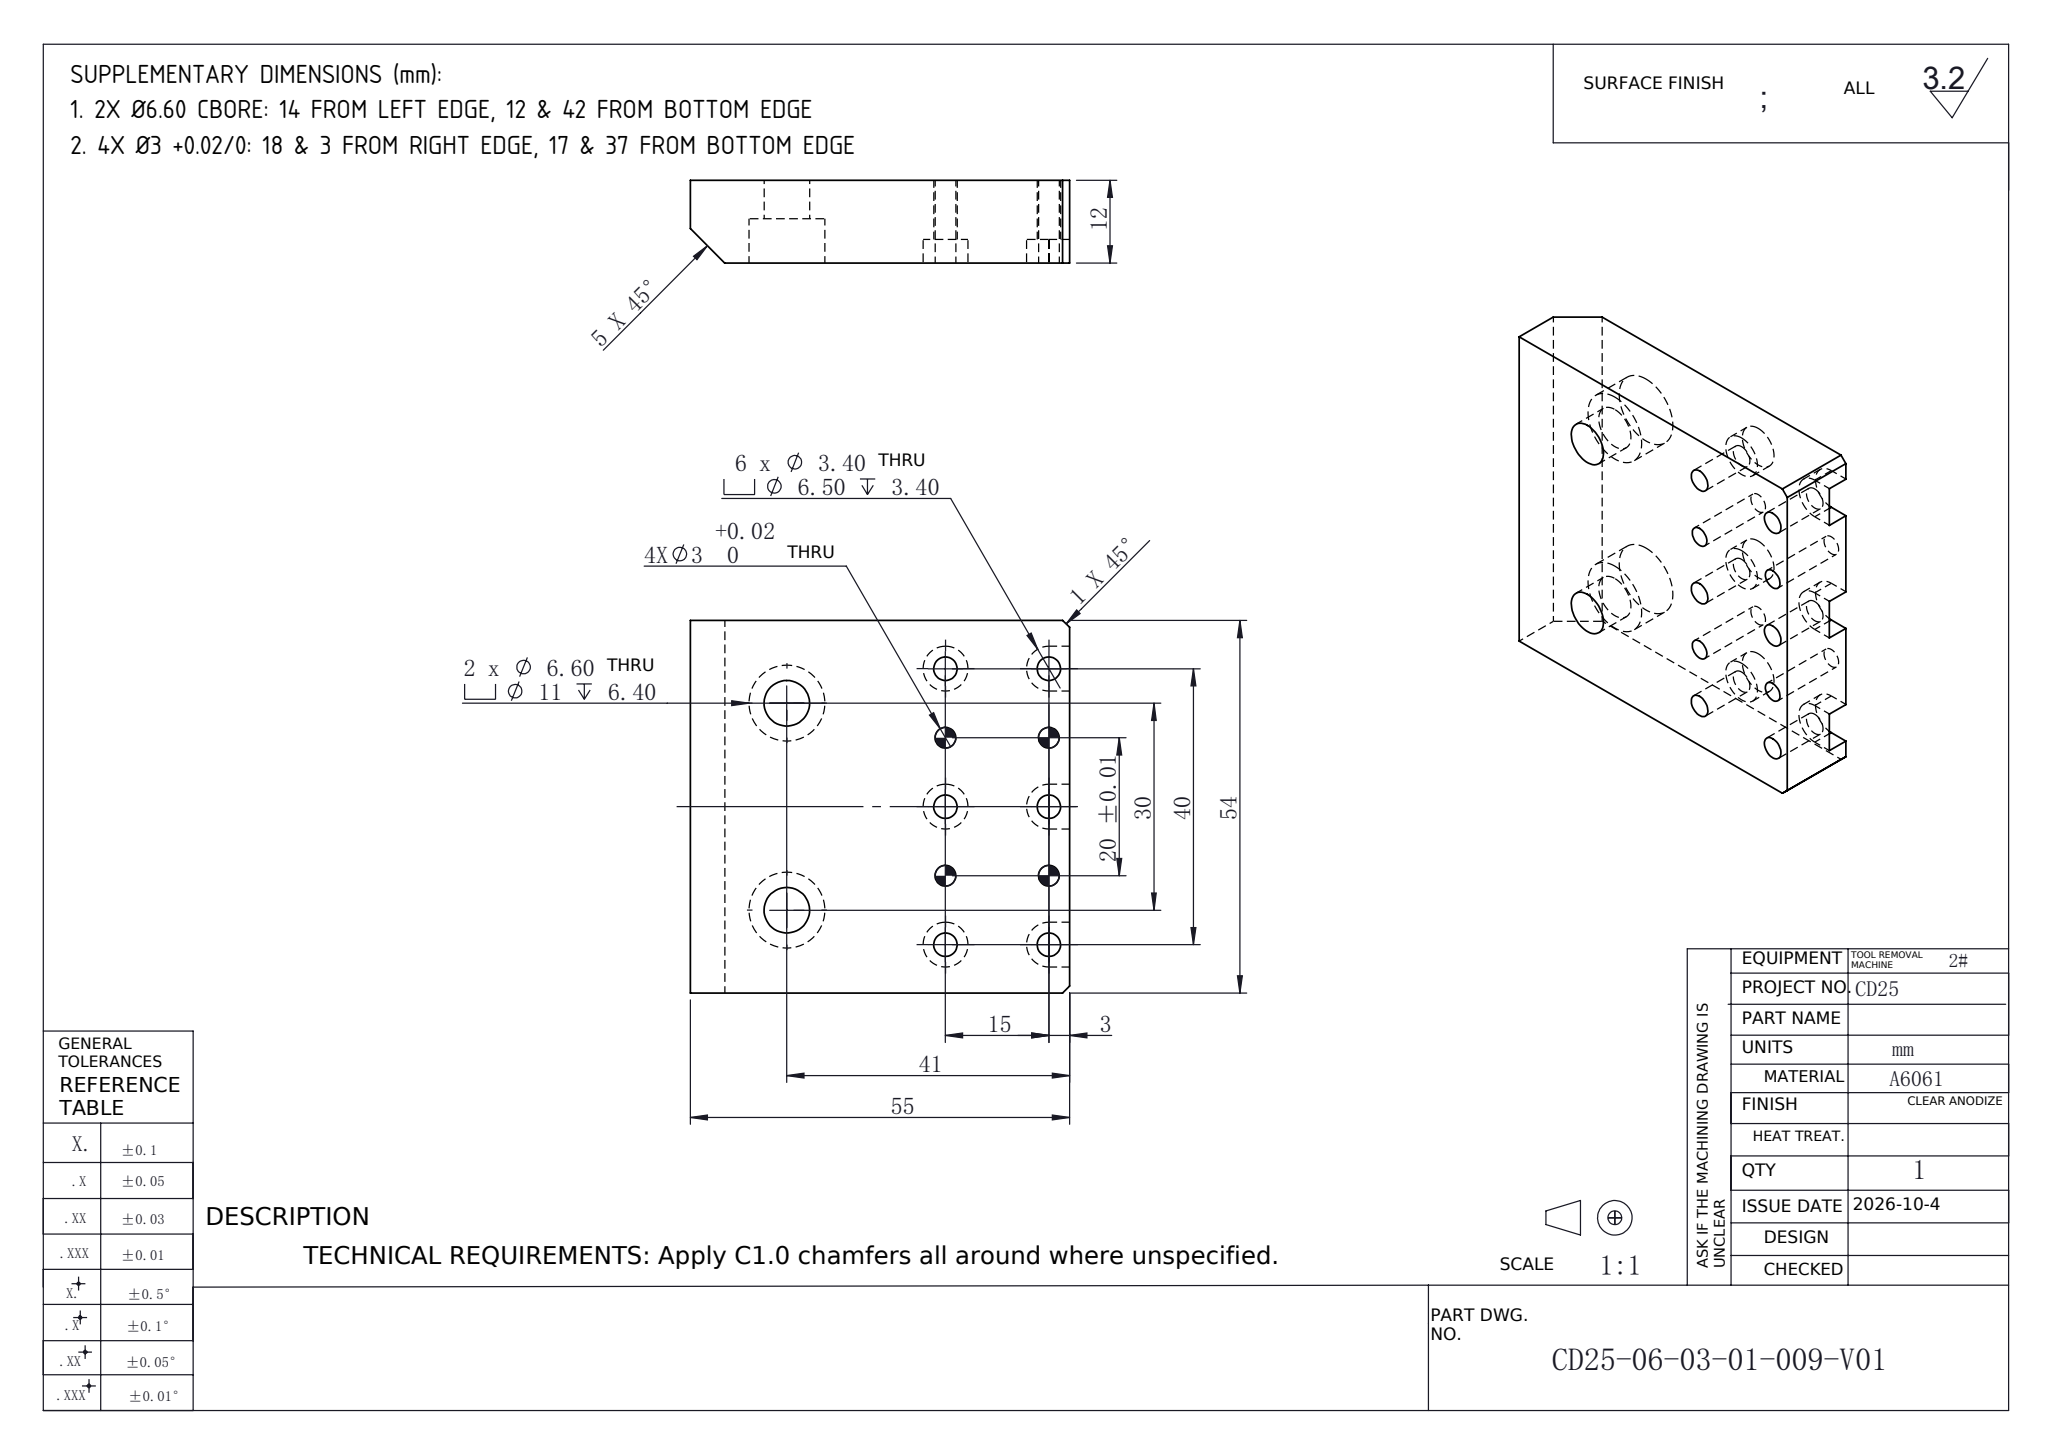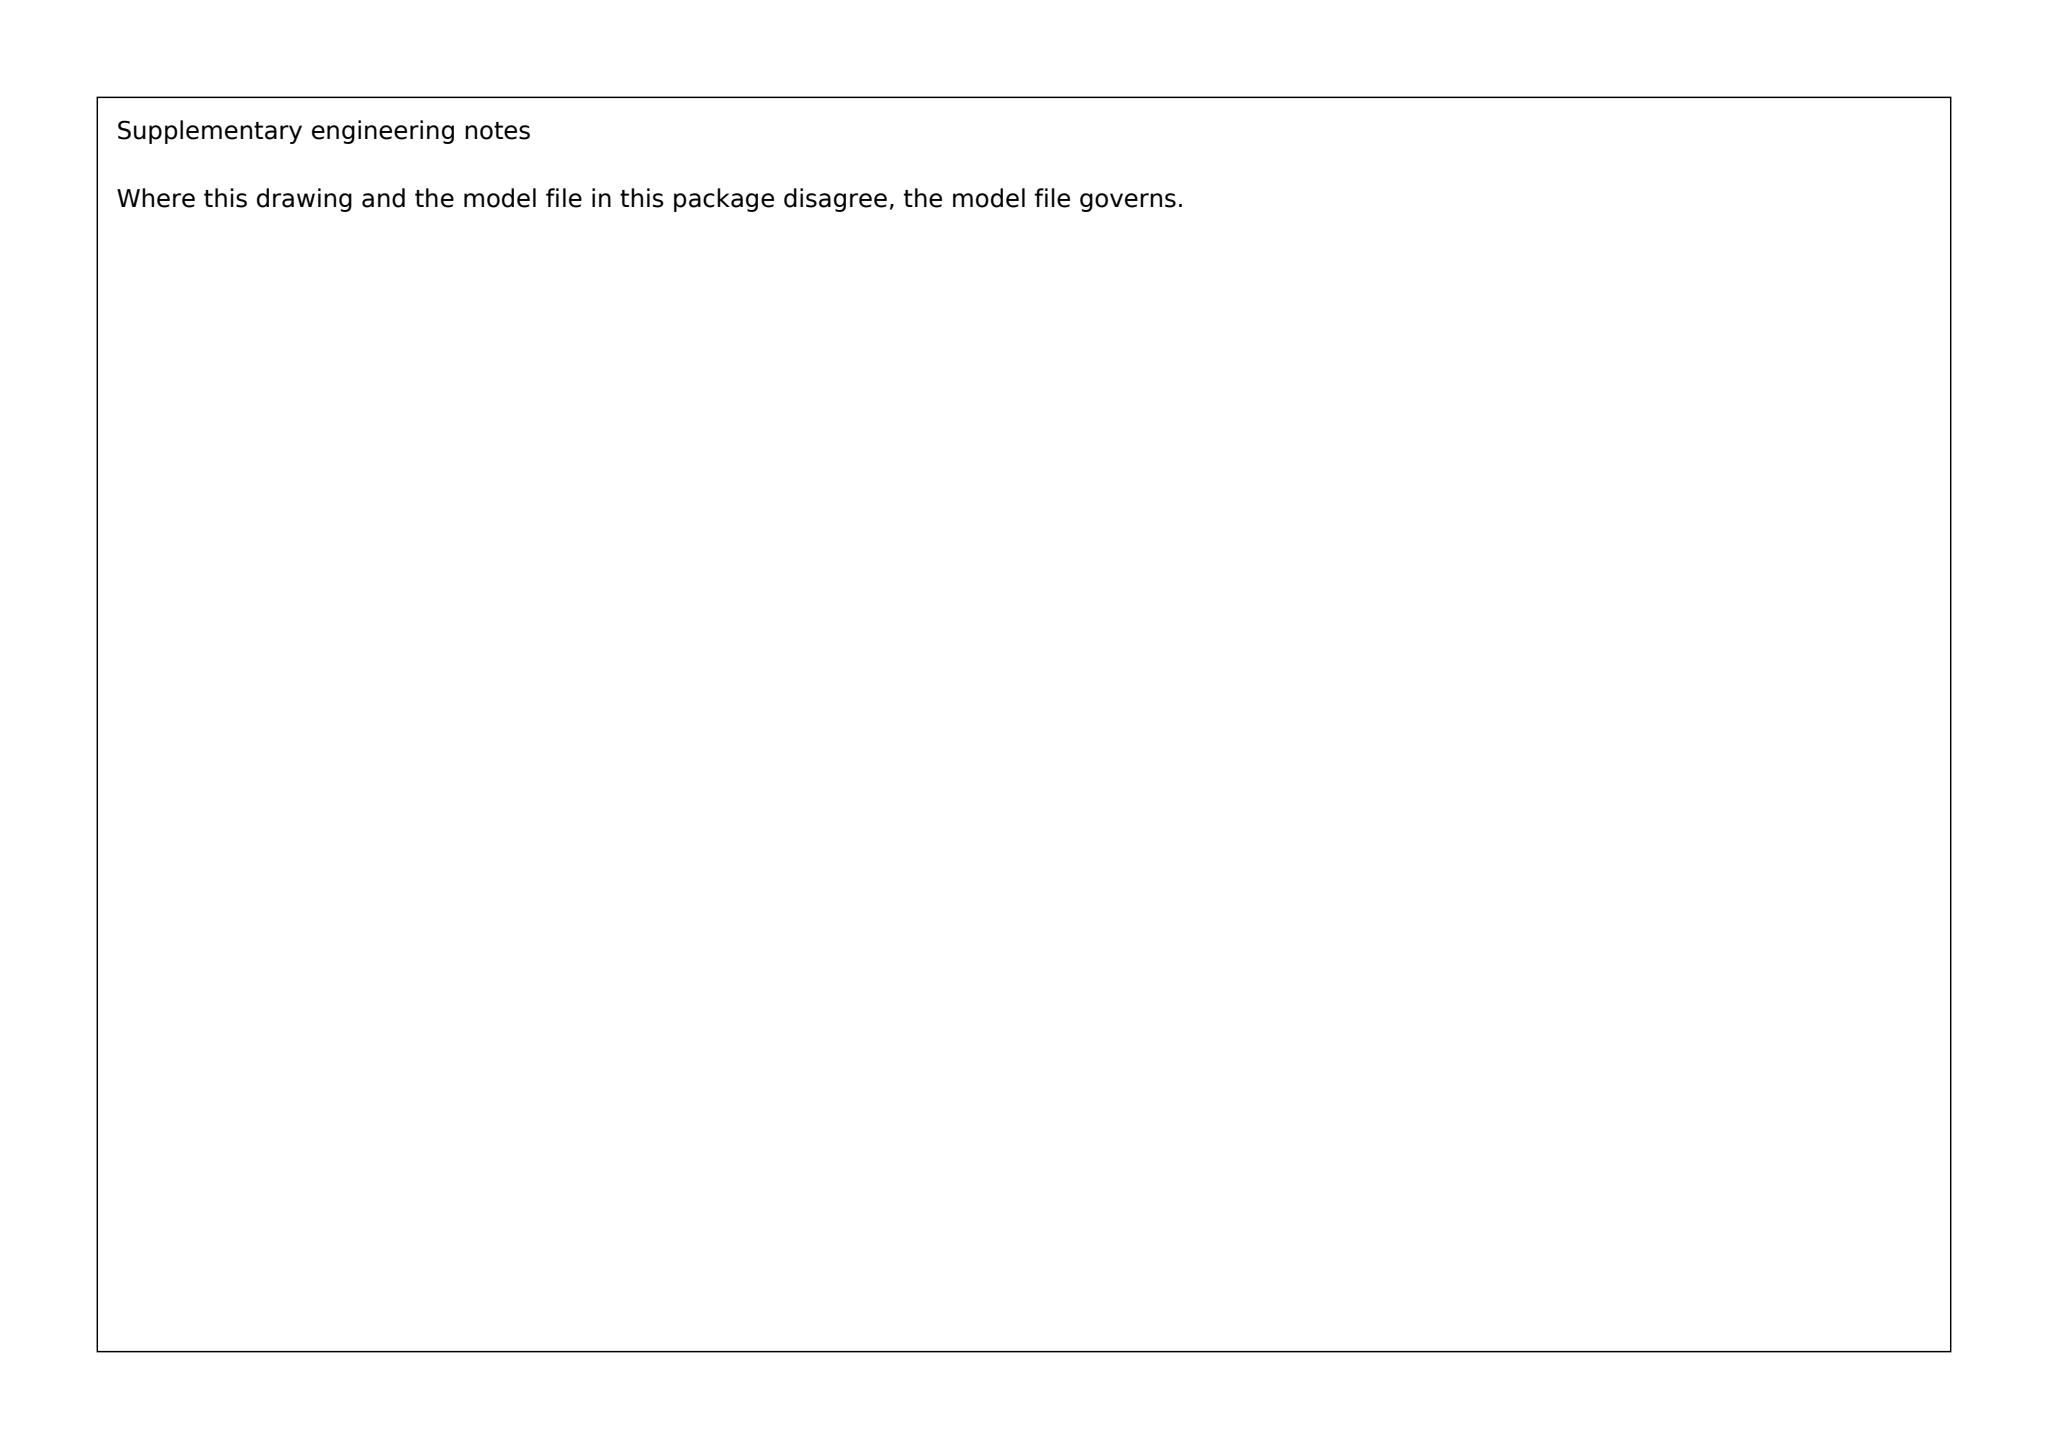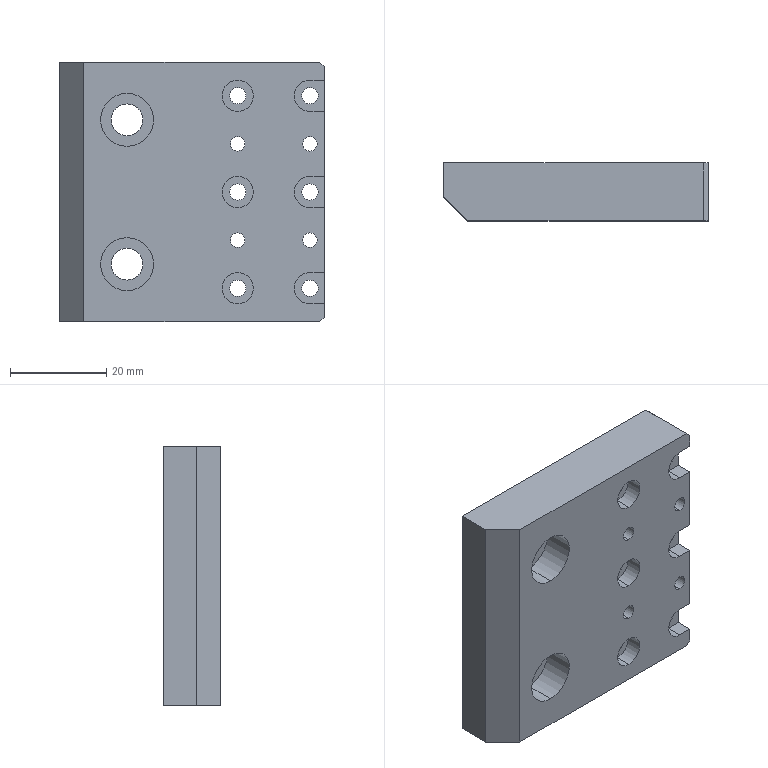Part | SolidWorks | mm | 1 solid | 60 faces | box 55 x 12 x 54 mm | volume 31839 mm3 | cylinder 37 | plane 23 | commonest cylinder face diameters 3.4 x12 6.5 x9 3 x8 11 x4 6.6 x4
build123d program:
from build123d import *

# Parameters (mm, degrees)
SKETCH1_W                                       = 55
SKETCH1_H                                       = 54
BOSS_EXTRUDE1_DEPTH                             = 6
M6_HEX_SOCKET_HEAD_CAP_SCREW_CBORE1_D           = 6.6
M6_HEX_SOCKET_HEAD_CAP_SCREW_CBORE1_CBORE_D     = 11
M6_HEX_SOCKET_HEAD_CAP_SCREW_CBORE1_CBORE_DEPTH = 6.4
M3_HEX_SOCKET_HEAD_CAP_SCREW_CBORE1_D           = 3.4
M3_HEX_SOCKET_HEAD_CAP_SCREW_CBORE1_CBORE_D     = 6.5
M3_HEX_SOCKET_HEAD_CAP_SCREW_CBORE1_CBORE_DEPTH = 3.4
F_3_0MM_DOWEL_PIN_HOLE1_D                       = 3
CUT_EXTRUDE1_DEPTH                              = 3.4
CHAMFER1_SIZE                                   = 1
CHAMFER2_SIZE                                   = 5


with BuildPart() as part:
    # Sketch1 → Boss-Extrude1 (new, symmetric)
    with BuildSketch(Plane(origin=(0, 0, 0), x_dir=(1, 0, 0), z_dir=(0, 1, 0))):
        Rectangle(SKETCH1_W, SKETCH1_H)
    extrude(amount=BOSS_EXTRUDE1_DEPTH, both=True)

    # M6 Hex Socket Head Cap Screw CBORE1 (through all)
    with Locations(Plane(origin=(0, -6, 0), x_dir=(-1, 0, 0), z_dir=(0, -1, 0))):
        with Locations((13.5, 15), (13.5, -15)):
            CounterBoreHole(M6_HEX_SOCKET_HEAD_CAP_SCREW_CBORE1_D / 2, M6_HEX_SOCKET_HEAD_CAP_SCREW_CBORE1_CBORE_D / 2, M6_HEX_SOCKET_HEAD_CAP_SCREW_CBORE1_CBORE_DEPTH)

    # M3 Hex Socket Head Cap Screw CBORE1 (through all)
    with Locations(Plane(origin=(0, -6, 0), x_dir=(-1, 0, 0), z_dir=(0, -1, 0))):
        with Locations((-24.5, -20), (-9.5, -20), (-9.5, 0), (-24.5, 0), (-24.5, 20), (-9.5, 20)):
            CounterBoreHole(M3_HEX_SOCKET_HEAD_CAP_SCREW_CBORE1_D / 2, M3_HEX_SOCKET_HEAD_CAP_SCREW_CBORE1_CBORE_D / 2, M3_HEX_SOCKET_HEAD_CAP_SCREW_CBORE1_CBORE_DEPTH)

    # 3.0mm Dowel Pin Hole1 (through all)
    with Locations(Plane(origin=(0, -6, 0), x_dir=(-1, 0, 0), z_dir=(0, -1, 0))):
        with Locations((-24.5, 10), (-9.5, 10), (-9.5, -10), (-24.5, -10)):
            Hole(F_3_0MM_DOWEL_PIN_HOLE1_D / 2)

    # Sketch8 → Cut-Extrude1 (cut)
    with BuildSketch(Plane.XZ.offset(6)):
        with BuildLine():
            Line((24.5, 23.25), (27.5, 23.25))
            ThreePointArc((27.5, 23.25), (30.75, 20), (27.5, 16.75))
            Line((27.5, 16.75), (24.5, 16.75))
            ThreePointArc((24.5, 16.75), (21.25, 20), (24.5, 23.25))
        make_face()
        with BuildLine():
            Line((24.5, -23.25), (27.5, -23.25))
            ThreePointArc((27.5, -23.25), (30.75, -20), (27.5, -16.75))
            Line((27.5, -16.75), (24.5, -16.75))
            ThreePointArc((24.5, -16.75), (21.25, -20), (24.5, -23.25))
        make_face()
        with BuildLine():
            Line((24.5, 3.25), (27.5, 3.25))
            ThreePointArc((27.5, 3.25), (30.75, 0), (27.5, -3.25))
            Line((27.5, -3.25), (24.5, -3.25))
            ThreePointArc((24.5, -3.25), (21.25, 0), (24.5, 3.25))
        make_face()
    extrude(amount=-CUT_EXTRUDE1_DEPTH, mode=Mode.SUBTRACT)

    # Chamfer1
    chamfer1_edges = [part.edges().sort_by_distance(p)[0] for p in [
        (27.5, 0, 27),
        (27.5, 0, -27),
    ]]
    chamfer(chamfer1_edges, length=CHAMFER1_SIZE)

    # Chamfer2
    chamfer2_edges = [part.edges().sort_by_distance(p)[0] for p in [
        (-27.5, -6, 0),
    ]]
    chamfer(chamfer2_edges, length=CHAMFER2_SIZE)


solid = part.part